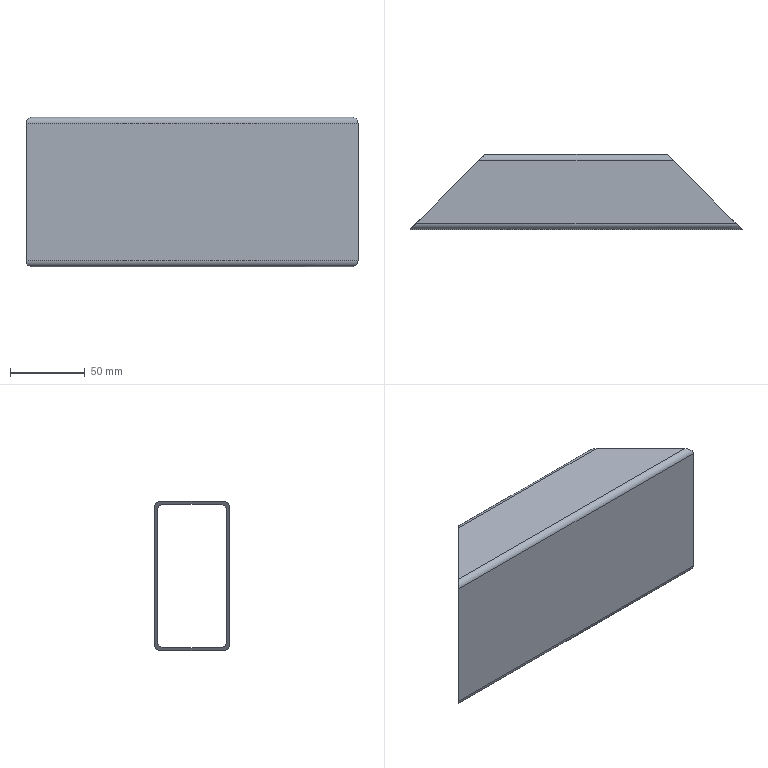Component | NX | SLID_FRAME_BEAM3_2 | 1 solid | 18 faces | volume 100448 mm3 | plane 10 | cylinder 8 | commonest cylinder face diameters 8 x8